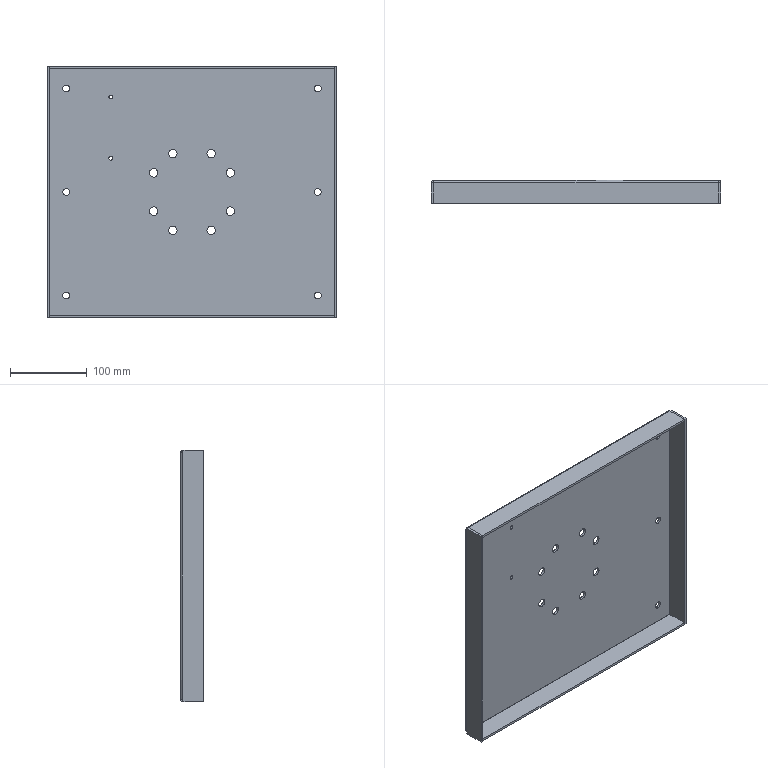Component | SolidWorks | CCD02LiftingBasePlate-1 | 1 solid | 78 faces | volume 478612 mm3 | cylinder 40 | plane 30 | spline 8 | commonest cylinder face diameters 11 x16 9 x12 5 x4 6.4 x4 0.4 x4